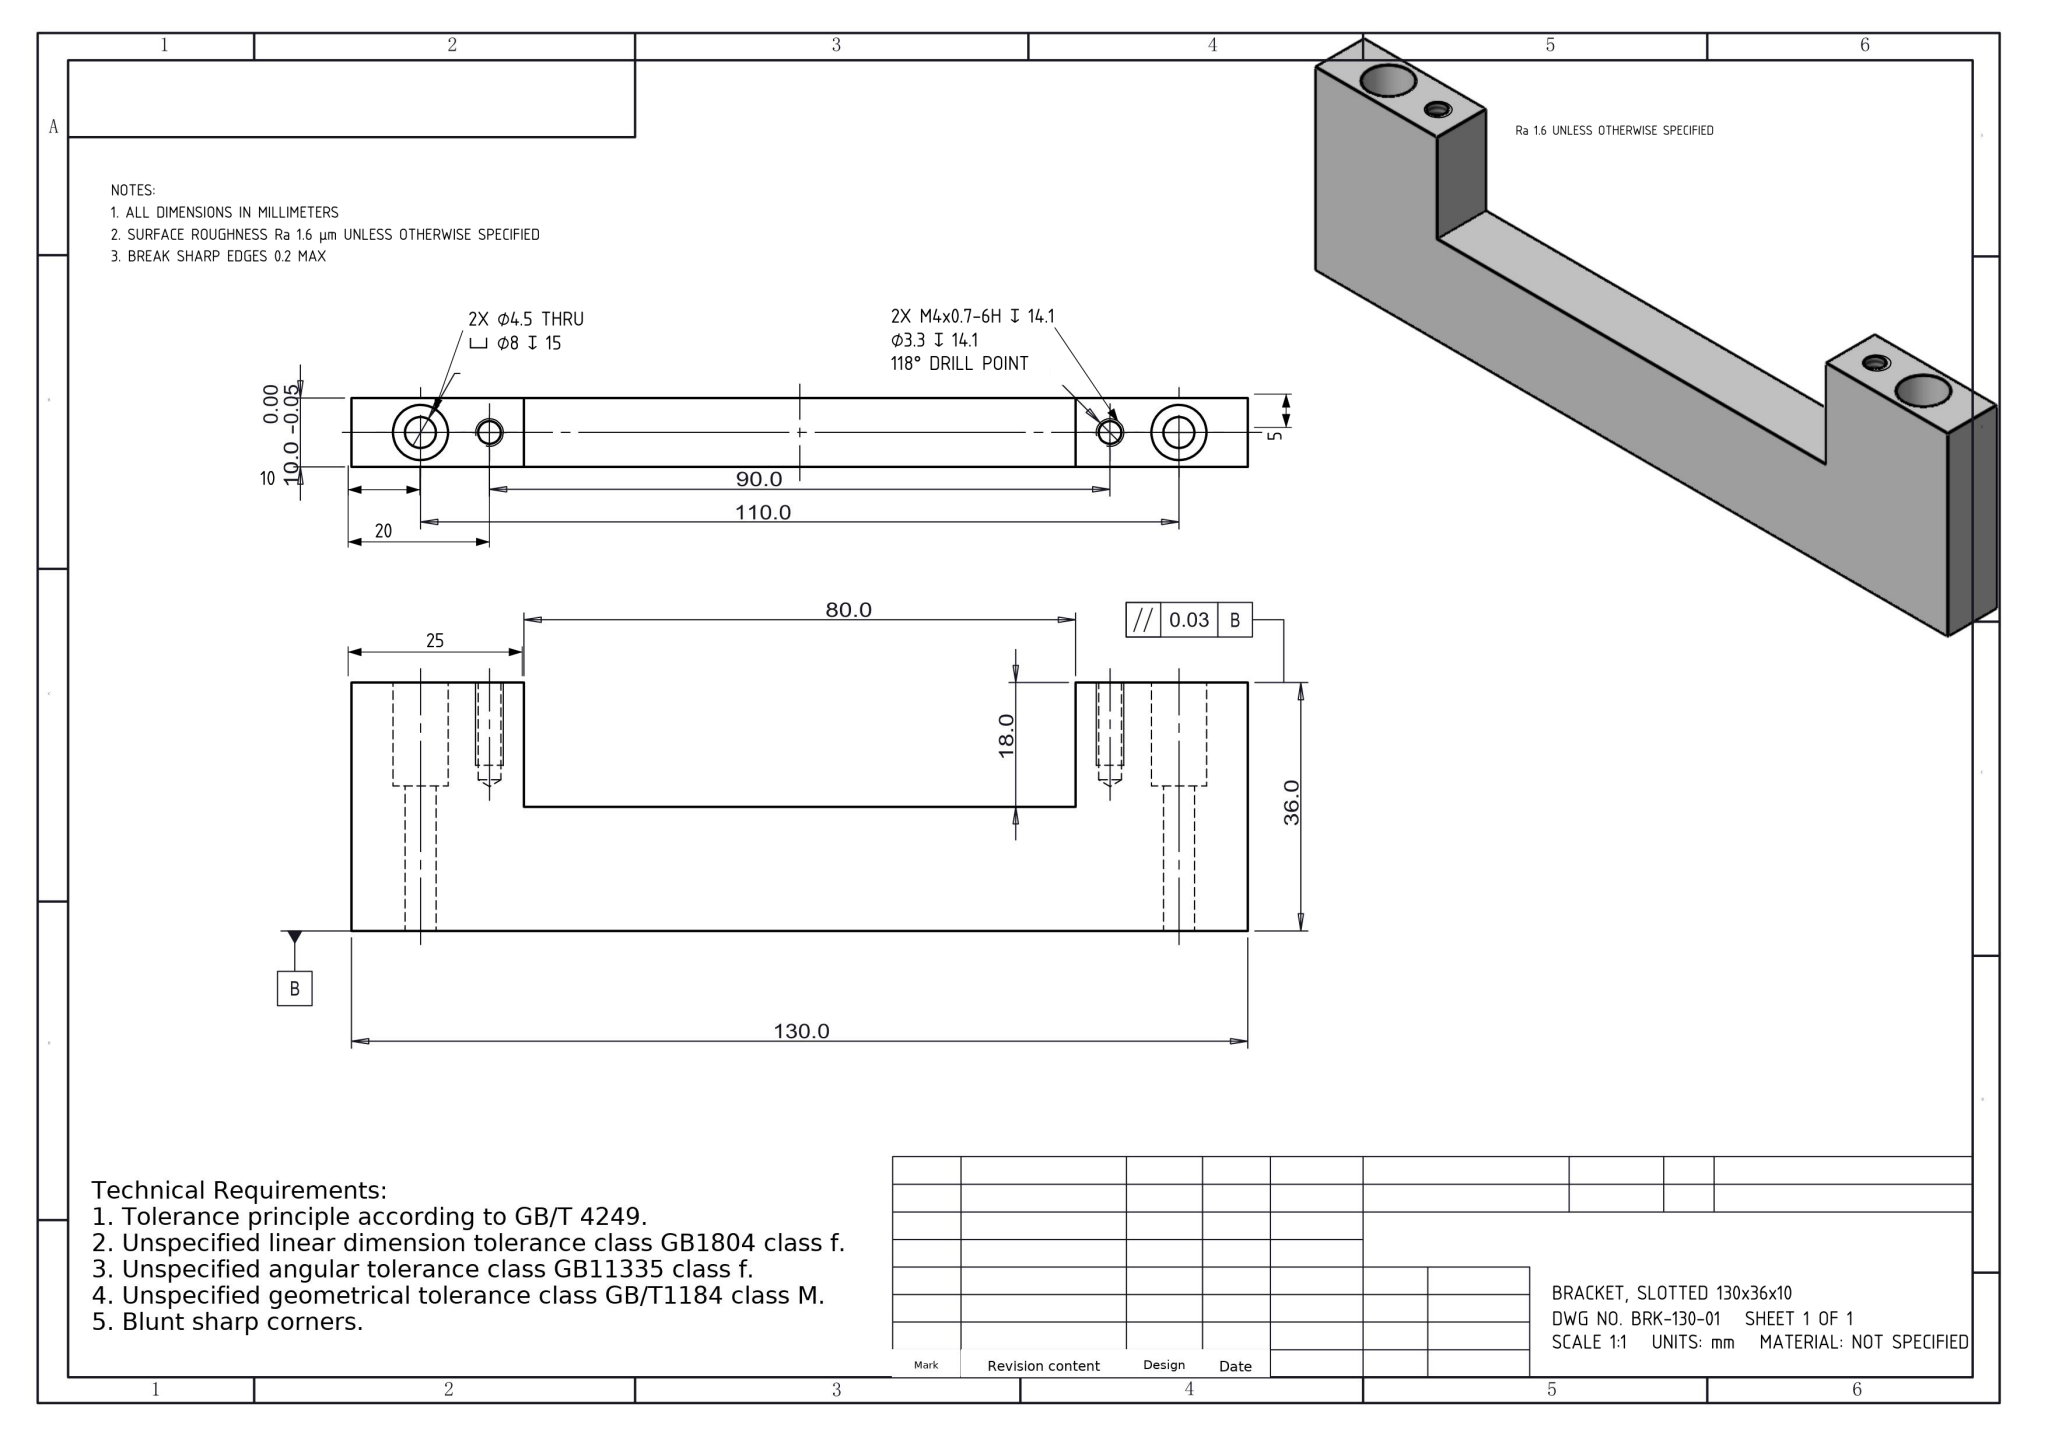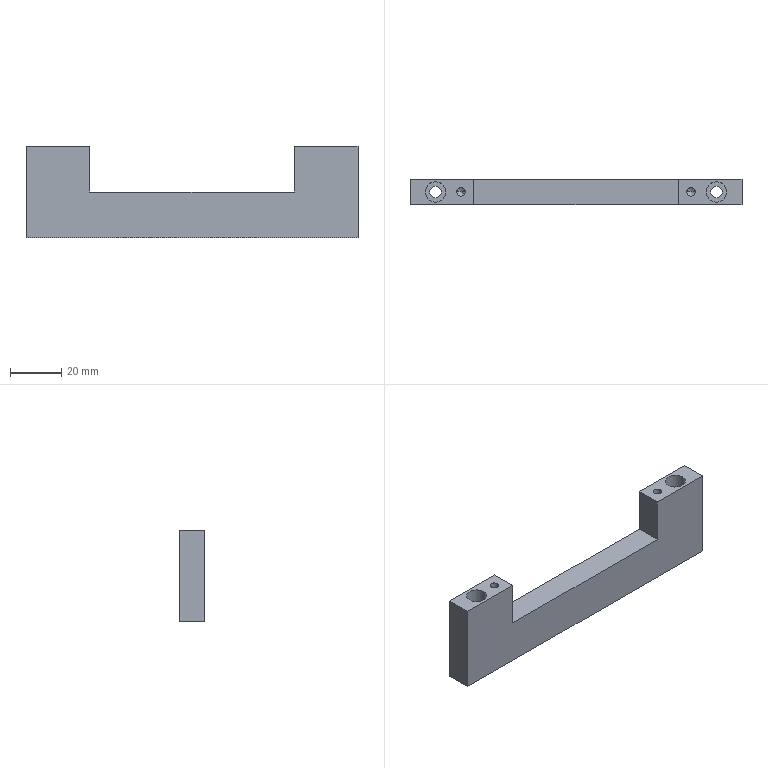Part | NX | mm | 1 solid | 28 faces | box 130 x 10 x 36 mm | volume 29977 mm3 | cylinder 12 | plane 12 | cone 4 | commonest cylinder face diameters 8 x4 4.5 x4 3.3 x4
STEP:
#1=COLOUR_RGB('',0.7529,0.7529,0.7529);
#2=FILL_AREA_STYLE_COLOUR('',#1);
#3=FILL_AREA_STYLE('',(#2));
#4=SURFACE_STYLE_FILL_AREA(#3);
#5=SURFACE_SIDE_STYLE('',(#4));
#6=SURFACE_STYLE_USAGE(.BOTH.,#5);
#7=PRESENTATION_STYLE_ASSIGNMENT((#6));
#8=CARTESIAN_POINT('',(51.,0.,21.));
#9=VERTEX_POINT('',#8);
#10=CARTESIAN_POINT('',(59.,0.,21.));
#11=VERTEX_POINT('',#10);
#12=CARTESIAN_POINT('',(55.,0.,21.));
#13=DIRECTION('',(0.,0.,1.));
#14=DIRECTION('',(1.,0.,0.));
#15=AXIS2_PLACEMENT_3D('',#12,#13,#14);
#16=CIRCLE('',#15,4.);
#17=EDGE_CURVE('',#9,#11,#16,.T.);
#18=ORIENTED_EDGE('',*,*,#17,.F.);
#19=CARTESIAN_POINT('',(51.,0.,36.));
#20=VERTEX_POINT('',#19);
#21=CARTESIAN_POINT('',(51.,0.,36.));
#22=DIRECTION('',(0.,0.,1.));
#23=VECTOR('',#22,1000.);
#24=LINE('',#21,#23);
#25=EDGE_CURVE('',#9,#20,#24,.T.);
#26=ORIENTED_EDGE('',*,*,#25,.T.);
#27=CARTESIAN_POINT('',(59.,0.,36.));
#28=VERTEX_POINT('',#27);
#29=CARTESIAN_POINT('',(55.,0.,36.));
#30=DIRECTION('',(0.,0.,1.));
#31=DIRECTION('',(1.,0.,0.));
#32=AXIS2_PLACEMENT_3D('',#29,#30,#31);
#33=CIRCLE('',#32,4.);
#34=EDGE_CURVE('',#20,#28,#33,.T.);
#35=ORIENTED_EDGE('',*,*,#34,.T.);
#36=CARTESIAN_POINT('',(59.,0.,36.));
#37=DIRECTION('',(0.,0.,1.));
#38=VECTOR('',#37,1000.);
#39=LINE('',#36,#38);
#40=EDGE_CURVE('',#11,#28,#39,.T.);
#41=ORIENTED_EDGE('',*,*,#40,.F.);
#42=EDGE_LOOP('',(#18,#26,#35,#41));
#43=FACE_OUTER_BOUND('',#42,.T.);
#44=CARTESIAN_POINT('',(55.,0.,36.));
#45=DIRECTION('',(0.,0.,1.));
#46=DIRECTION('',(1.,0.,0.));
#47=AXIS2_PLACEMENT_3D('',#44,#45,#46);
#48=CYLINDRICAL_SURFACE('',#47,4.);
#49=ADVANCED_FACE('',(#43),#48,.F.);
#50=CARTESIAN_POINT('',(52.75,0.,0.));
#51=VERTEX_POINT('',#50);
#52=CARTESIAN_POINT('',(57.25,0.,0.));
#53=VERTEX_POINT('',#52);
#54=CARTESIAN_POINT('',(55.,0.,0.));
#55=DIRECTION('',(0.,0.,1.));
#56=DIRECTION('',(1.,0.,0.));
#57=AXIS2_PLACEMENT_3D('',#54,#55,#56);
#58=CIRCLE('',#57,2.25);
#59=EDGE_CURVE('',#51,#53,#58,.T.);
#60=ORIENTED_EDGE('',*,*,#59,.F.);
#61=CARTESIAN_POINT('',(52.75,0.,21.));
#62=VERTEX_POINT('',#61);
#63=CARTESIAN_POINT('',(52.75,0.,36.));
#64=DIRECTION('',(0.,0.,1.));
#65=VECTOR('',#64,1000.);
#66=LINE('',#63,#65);
#67=EDGE_CURVE('',#51,#62,#66,.T.);
#68=ORIENTED_EDGE('',*,*,#67,.T.);
#69=CARTESIAN_POINT('',(57.25,0.,21.));
#70=VERTEX_POINT('',#69);
#71=CARTESIAN_POINT('',(55.,0.,21.));
#72=DIRECTION('',(0.,0.,1.));
#73=DIRECTION('',(1.,0.,0.));
#74=AXIS2_PLACEMENT_3D('',#71,#72,#73);
#75=CIRCLE('',#74,2.25);
#76=EDGE_CURVE('',#62,#70,#75,.T.);
#77=ORIENTED_EDGE('',*,*,#76,.T.);
#78=CARTESIAN_POINT('',(57.25,0.,36.));
#79=DIRECTION('',(0.,0.,1.));
#80=VECTOR('',#79,1000.);
#81=LINE('',#78,#80);
#82=EDGE_CURVE('',#53,#70,#81,.T.);
#83=ORIENTED_EDGE('',*,*,#82,.F.);
#84=EDGE_LOOP('',(#60,#68,#77,#83));
#85=FACE_OUTER_BOUND('',#84,.T.);
#86=CARTESIAN_POINT('',(55.,0.,36.));
#87=DIRECTION('',(0.,0.,1.));
#88=DIRECTION('',(1.,0.,0.));
#89=AXIS2_PLACEMENT_3D('',#86,#87,#88);
#90=CYLINDRICAL_SURFACE('',#89,2.25);
#91=ADVANCED_FACE('',(#85),#90,.F.);
#92=CARTESIAN_POINT('',(-59.,0.,21.));
#93=VERTEX_POINT('',#92);
#94=CARTESIAN_POINT('',(-51.,0.,21.));
#95=VERTEX_POINT('',#94);
#96=CARTESIAN_POINT('',(-55.,0.,21.));
#97=DIRECTION('',(0.,0.,1.));
#98=DIRECTION('',(1.,0.,0.));
#99=AXIS2_PLACEMENT_3D('',#96,#97,#98);
#100=CIRCLE('',#99,4.);
#101=EDGE_CURVE('',#93,#95,#100,.T.);
#102=ORIENTED_EDGE('',*,*,#101,.F.);
#103=CARTESIAN_POINT('',(-59.,0.,36.));
#104=VERTEX_POINT('',#103);
#105=CARTESIAN_POINT('',(-59.,0.,36.));
#106=DIRECTION('',(0.,0.,1.));
#107=VECTOR('',#106,1000.);
#108=LINE('',#105,#107);
#109=EDGE_CURVE('',#93,#104,#108,.T.);
#110=ORIENTED_EDGE('',*,*,#109,.T.);
#111=CARTESIAN_POINT('',(-51.,0.,36.));
#112=VERTEX_POINT('',#111);
#113=CARTESIAN_POINT('',(-55.,0.,36.));
#114=DIRECTION('',(0.,0.,1.));
#115=DIRECTION('',(1.,0.,0.));
#116=AXIS2_PLACEMENT_3D('',#113,#114,#115);
#117=CIRCLE('',#116,4.);
#118=EDGE_CURVE('',#104,#112,#117,.T.);
#119=ORIENTED_EDGE('',*,*,#118,.T.);
#120=CARTESIAN_POINT('',(-51.,0.,36.));
#121=DIRECTION('',(0.,0.,1.));
#122=VECTOR('',#121,1000.);
#123=LINE('',#120,#122);
#124=EDGE_CURVE('',#95,#112,#123,.T.);
#125=ORIENTED_EDGE('',*,*,#124,.F.);
#126=EDGE_LOOP('',(#102,#110,#119,#125));
#127=FACE_OUTER_BOUND('',#126,.T.);
#128=CARTESIAN_POINT('',(-55.,0.,36.));
#129=DIRECTION('',(0.,0.,1.));
#130=DIRECTION('',(1.,0.,0.));
#131=AXIS2_PLACEMENT_3D('',#128,#129,#130);
#132=CYLINDRICAL_SURFACE('',#131,4.);
#133=ADVANCED_FACE('',(#127),#132,.F.);
#134=CARTESIAN_POINT('',(-57.25,0.,0.));
#135=VERTEX_POINT('',#134);
#136=CARTESIAN_POINT('',(-52.75,0.,0.));
#137=VERTEX_POINT('',#136);
#138=CARTESIAN_POINT('',(-55.,0.,0.));
#139=DIRECTION('',(0.,0.,1.));
#140=DIRECTION('',(1.,0.,0.));
#141=AXIS2_PLACEMENT_3D('',#138,#139,#140);
#142=CIRCLE('',#141,2.25);
#143=EDGE_CURVE('',#135,#137,#142,.T.);
#144=ORIENTED_EDGE('',*,*,#143,.F.);
#145=CARTESIAN_POINT('',(-57.25,0.,21.));
#146=VERTEX_POINT('',#145);
#147=CARTESIAN_POINT('',(-57.25,0.,36.));
#148=DIRECTION('',(0.,0.,1.));
#149=VECTOR('',#148,1000.);
#150=LINE('',#147,#149);
#151=EDGE_CURVE('',#135,#146,#150,.T.);
#152=ORIENTED_EDGE('',*,*,#151,.T.);
#153=CARTESIAN_POINT('',(-52.75,0.,21.));
#154=VERTEX_POINT('',#153);
#155=CARTESIAN_POINT('',(-55.,0.,21.));
#156=DIRECTION('',(0.,0.,1.));
#157=DIRECTION('',(1.,0.,0.));
#158=AXIS2_PLACEMENT_3D('',#155,#156,#157);
#159=CIRCLE('',#158,2.25);
#160=EDGE_CURVE('',#146,#154,#159,.T.);
#161=ORIENTED_EDGE('',*,*,#160,.T.);
#162=CARTESIAN_POINT('',(-52.75,0.,36.));
#163=DIRECTION('',(0.,0.,1.));
#164=VECTOR('',#163,1000.);
#165=LINE('',#162,#164);
#166=EDGE_CURVE('',#137,#154,#165,.T.);
#167=ORIENTED_EDGE('',*,*,#166,.F.);
#168=EDGE_LOOP('',(#144,#152,#161,#167));
#169=FACE_OUTER_BOUND('',#168,.T.);
#170=CARTESIAN_POINT('',(-55.,0.,36.));
#171=DIRECTION('',(0.,0.,1.));
#172=DIRECTION('',(1.,0.,0.));
#173=AXIS2_PLACEMENT_3D('',#170,#171,#172);
#174=CYLINDRICAL_SURFACE('',#173,2.25);
#175=ADVANCED_FACE('',(#169),#174,.F.);
#176=CARTESIAN_POINT('',(43.35,0.,21.9));
#177=VERTEX_POINT('',#176);
#178=CARTESIAN_POINT('',(46.65,0.,21.9));
#179=VERTEX_POINT('',#178);
#180=CARTESIAN_POINT('',(45.,0.,21.9));
#181=DIRECTION('',(0.,0.,1.));
#182=DIRECTION('',(1.,0.,0.));
#183=AXIS2_PLACEMENT_3D('',#180,#181,#182);
#184=CIRCLE('',#183,1.65);
#185=EDGE_CURVE('',#177,#179,#184,.T.);
#186=ORIENTED_EDGE('',*,*,#185,.F.);
#187=CARTESIAN_POINT('',(43.35,0.,36.));
#188=VERTEX_POINT('',#187);
#189=CARTESIAN_POINT('',(43.35,0.,36.));
#190=DIRECTION('',(0.,0.,1.));
#191=VECTOR('',#190,1000.);
#192=LINE('',#189,#191);
#193=EDGE_CURVE('',#177,#188,#192,.T.);
#194=ORIENTED_EDGE('',*,*,#193,.T.);
#195=CARTESIAN_POINT('',(46.65,0.,36.));
#196=VERTEX_POINT('',#195);
#197=CARTESIAN_POINT('',(45.,0.,36.));
#198=DIRECTION('',(0.,0.,1.));
#199=DIRECTION('',(1.,0.,0.));
#200=AXIS2_PLACEMENT_3D('',#197,#198,#199);
#201=CIRCLE('',#200,1.65);
#202=EDGE_CURVE('',#188,#196,#201,.T.);
#203=ORIENTED_EDGE('',*,*,#202,.T.);
#204=CARTESIAN_POINT('',(46.65,0.,36.));
#205=DIRECTION('',(0.,0.,1.));
#206=VECTOR('',#205,1000.);
#207=LINE('',#204,#206);
#208=EDGE_CURVE('',#179,#196,#207,.T.);
#209=ORIENTED_EDGE('',*,*,#208,.F.);
#210=EDGE_LOOP('',(#186,#194,#203,#209));
#211=FACE_OUTER_BOUND('',#210,.T.);
#212=CARTESIAN_POINT('',(45.,0.,36.));
#213=DIRECTION('',(0.,0.,1.));
#214=DIRECTION('',(1.,0.,0.));
#215=AXIS2_PLACEMENT_3D('',#212,#213,#214);
#216=CYLINDRICAL_SURFACE('',#215,1.65);
#217=ADVANCED_FACE('',(#211),#216,.F.);
#218=CARTESIAN_POINT('',(45.,0.,20.909));
#219=VERTEX_POINT('',#218);
#220=CARTESIAN_POINT('',(46.65,0.,21.9));
#221=DIRECTION('',(0.8572,0.,0.515));
#222=VECTOR('',#221,1000.);
#223=LINE('',#220,#222);
#224=EDGE_CURVE('',#219,#179,#223,.T.);
#225=ORIENTED_EDGE('',*,*,#224,.F.);
#226=CARTESIAN_POINT('',(43.35,0.,21.9));
#227=DIRECTION('',(-0.8572,0.,0.515));
#228=VECTOR('',#227,1000.);
#229=LINE('',#226,#228);
#230=EDGE_CURVE('',#219,#177,#229,.T.);
#231=ORIENTED_EDGE('',*,*,#230,.T.);
#232=ORIENTED_EDGE('',*,*,#185,.T.);
#233=EDGE_LOOP('',(#225,#231,#232));
#234=FACE_OUTER_BOUND('',#233,.T.);
#235=CARTESIAN_POINT('',(45.,0.,21.9));
#236=DIRECTION('',(0.,0.,1.));
#237=DIRECTION('',(1.,0.,0.));
#238=AXIS2_PLACEMENT_3D('',#235,#236,#237);
#239=CONICAL_SURFACE('',#238,1.65,1.03);
#240=ADVANCED_FACE('',(#234),#239,.F.);
#241=CARTESIAN_POINT('',(-46.65,0.,21.9));
#242=VERTEX_POINT('',#241);
#243=CARTESIAN_POINT('',(-43.35,0.,21.9));
#244=VERTEX_POINT('',#243);
#245=CARTESIAN_POINT('',(-45.,0.,21.9));
#246=DIRECTION('',(0.,0.,1.));
#247=DIRECTION('',(1.,0.,0.));
#248=AXIS2_PLACEMENT_3D('',#245,#246,#247);
#249=CIRCLE('',#248,1.65);
#250=EDGE_CURVE('',#242,#244,#249,.T.);
#251=ORIENTED_EDGE('',*,*,#250,.F.);
#252=CARTESIAN_POINT('',(-46.65,0.,36.));
#253=VERTEX_POINT('',#252);
#254=CARTESIAN_POINT('',(-46.65,0.,36.));
#255=DIRECTION('',(0.,0.,1.));
#256=VECTOR('',#255,1000.);
#257=LINE('',#254,#256);
#258=EDGE_CURVE('',#242,#253,#257,.T.);
#259=ORIENTED_EDGE('',*,*,#258,.T.);
#260=CARTESIAN_POINT('',(-43.35,0.,36.));
#261=VERTEX_POINT('',#260);
#262=CARTESIAN_POINT('',(-45.,0.,36.));
#263=DIRECTION('',(0.,0.,1.));
#264=DIRECTION('',(1.,0.,0.));
#265=AXIS2_PLACEMENT_3D('',#262,#263,#264);
#266=CIRCLE('',#265,1.65);
#267=EDGE_CURVE('',#253,#261,#266,.T.);
#268=ORIENTED_EDGE('',*,*,#267,.T.);
#269=CARTESIAN_POINT('',(-43.35,0.,36.));
#270=DIRECTION('',(0.,0.,1.));
#271=VECTOR('',#270,1000.);
#272=LINE('',#269,#271);
#273=EDGE_CURVE('',#244,#261,#272,.T.);
#274=ORIENTED_EDGE('',*,*,#273,.F.);
#275=EDGE_LOOP('',(#251,#259,#268,#274));
#276=FACE_OUTER_BOUND('',#275,.T.);
#277=CARTESIAN_POINT('',(-45.,0.,36.));
#278=DIRECTION('',(0.,0.,1.));
#279=DIRECTION('',(1.,0.,0.));
#280=AXIS2_PLACEMENT_3D('',#277,#278,#279);
#281=CYLINDRICAL_SURFACE('',#280,1.65);
#282=ADVANCED_FACE('',(#276),#281,.F.);
#283=CARTESIAN_POINT('',(-45.,0.,20.909));
#284=VERTEX_POINT('',#283);
#285=CARTESIAN_POINT('',(-43.35,0.,21.9));
#286=DIRECTION('',(0.8572,0.,0.515));
#287=VECTOR('',#286,1000.);
#288=LINE('',#285,#287);
#289=EDGE_CURVE('',#284,#244,#288,.T.);
#290=ORIENTED_EDGE('',*,*,#289,.F.);
#291=CARTESIAN_POINT('',(-46.65,0.,21.9));
#292=DIRECTION('',(-0.8572,0.,0.515));
#293=VECTOR('',#292,1000.);
#294=LINE('',#291,#293);
#295=EDGE_CURVE('',#284,#242,#294,.T.);
#296=ORIENTED_EDGE('',*,*,#295,.T.);
#297=ORIENTED_EDGE('',*,*,#250,.T.);
#298=EDGE_LOOP('',(#290,#296,#297));
#299=FACE_OUTER_BOUND('',#298,.T.);
#300=CARTESIAN_POINT('',(-45.,0.,21.9));
#301=DIRECTION('',(0.,0.,1.));
#302=DIRECTION('',(1.,0.,0.));
#303=AXIS2_PLACEMENT_3D('',#300,#301,#302);
#304=CONICAL_SURFACE('',#303,1.65,1.03);
#305=ADVANCED_FACE('',(#299),#304,.F.);
#306=CARTESIAN_POINT('',(-40.,5.,36.));
#307=VERTEX_POINT('',#306);
#308=CARTESIAN_POINT('',(-40.,-5.,36.));
#309=VERTEX_POINT('',#308);
#310=CARTESIAN_POINT('',(-40.,5.,36.));
#311=DIRECTION('',(0.,-1.,0.));
#312=VECTOR('',#311,1000.);
#313=LINE('',#310,#312);
#314=EDGE_CURVE('',#307,#309,#313,.T.);
#315=ORIENTED_EDGE('',*,*,#314,.F.);
#316=CARTESIAN_POINT('',(-65.,5.,36.));
#317=VERTEX_POINT('',#316);
#318=CARTESIAN_POINT('',(-65.,5.,36.));
#319=DIRECTION('',(-1.,0.,0.));
#320=VECTOR('',#319,1000.);
#321=LINE('',#318,#320);
#322=EDGE_CURVE('',#307,#317,#321,.T.);
#323=ORIENTED_EDGE('',*,*,#322,.T.);
#324=CARTESIAN_POINT('',(-65.,-5.,36.));
#325=VERTEX_POINT('',#324);
#326=CARTESIAN_POINT('',(-65.,5.,36.));
#327=DIRECTION('',(0.,-1.,0.));
#328=VECTOR('',#327,1000.);
#329=LINE('',#326,#328);
#330=EDGE_CURVE('',#317,#325,#329,.T.);
#331=ORIENTED_EDGE('',*,*,#330,.T.);
#332=CARTESIAN_POINT('',(-65.,-5.,36.));
#333=DIRECTION('',(1.,0.,0.));
#334=VECTOR('',#333,1000.);
#335=LINE('',#332,#334);
#336=EDGE_CURVE('',#325,#309,#335,.T.);
#337=ORIENTED_EDGE('',*,*,#336,.T.);
#338=EDGE_LOOP('',(#315,#323,#331,#337));
#339=FACE_OUTER_BOUND('',#338,.T.);
#340=CARTESIAN_POINT('',(-45.,0.,36.));
#341=DIRECTION('',(0.,0.,1.));
#342=DIRECTION('',(1.,0.,0.));
#343=AXIS2_PLACEMENT_3D('',#340,#341,#342);
#344=CIRCLE('',#343,1.65);
#345=EDGE_CURVE('',#261,#253,#344,.T.);
#346=ORIENTED_EDGE('',*,*,#345,.F.);
#347=ORIENTED_EDGE('',*,*,#267,.F.);
#348=EDGE_LOOP('',(#346,#347));
#349=FACE_BOUND('',#348,.T.);
#350=CARTESIAN_POINT('',(-55.,0.,36.));
#351=DIRECTION('',(0.,0.,1.));
#352=DIRECTION('',(1.,0.,0.));
#353=AXIS2_PLACEMENT_3D('',#350,#351,#352);
#354=CIRCLE('',#353,4.);
#355=EDGE_CURVE('',#112,#104,#354,.T.);
#356=ORIENTED_EDGE('',*,*,#355,.F.);
#357=ORIENTED_EDGE('',*,*,#118,.F.);
#358=EDGE_LOOP('',(#356,#357));
#359=FACE_BOUND('',#358,.T.);
#360=CARTESIAN_POINT('',(65.,-5.,36.));
#361=DIRECTION('',(0.,0.,1.));
#362=DIRECTION('',(1.,0.,0.));
#363=AXIS2_PLACEMENT_3D('',#360,#361,#362);
#364=PLANE('',#363);
#365=ADVANCED_FACE('',(#339,#349,#359),#364,.T.);
#366=CARTESIAN_POINT('',(65.,-5.,0.));
#367=VERTEX_POINT('',#366);
#368=CARTESIAN_POINT('',(65.,5.,0.));
#369=VERTEX_POINT('',#368);
#370=CARTESIAN_POINT('',(65.,5.,0.));
#371=DIRECTION('',(0.,1.,0.));
#372=VECTOR('',#371,1000.);
#373=LINE('',#370,#372);
#374=EDGE_CURVE('',#367,#369,#373,.T.);
#375=ORIENTED_EDGE('',*,*,#374,.T.);
#376=CARTESIAN_POINT('',(65.,5.,36.));
#377=VERTEX_POINT('',#376);
#378=CARTESIAN_POINT('',(65.,5.,36.));
#379=DIRECTION('',(0.,0.,-1.));
#380=VECTOR('',#379,1000.);
#381=LINE('',#378,#380);
#382=EDGE_CURVE('',#377,#369,#381,.T.);
#383=ORIENTED_EDGE('',*,*,#382,.F.);
#384=CARTESIAN_POINT('',(65.,-5.,36.));
#385=VERTEX_POINT('',#384);
#386=CARTESIAN_POINT('',(65.,5.,36.));
#387=DIRECTION('',(0.,1.,0.));
#388=VECTOR('',#387,1000.);
#389=LINE('',#386,#388);
#390=EDGE_CURVE('',#385,#377,#389,.T.);
#391=ORIENTED_EDGE('',*,*,#390,.F.);
#392=CARTESIAN_POINT('',(65.,-5.,36.));
#393=DIRECTION('',(0.,0.,-1.));
#394=VECTOR('',#393,1000.);
#395=LINE('',#392,#394);
#396=EDGE_CURVE('',#385,#367,#395,.T.);
#397=ORIENTED_EDGE('',*,*,#396,.T.);
#398=EDGE_LOOP('',(#375,#383,#391,#397));
#399=FACE_OUTER_BOUND('',#398,.T.);
#400=CARTESIAN_POINT('',(65.,5.,36.));
#401=DIRECTION('',(-1.,0.,0.));
#402=DIRECTION('',(0.,0.,1.));
#403=AXIS2_PLACEMENT_3D('',#400,#401,#402);
#404=PLANE('',#403);
#405=ADVANCED_FACE('',(#399),#404,.F.);
#406=ORIENTED_EDGE('',*,*,#322,.F.);
#407=CARTESIAN_POINT('',(-40.,5.,18.));
#408=VERTEX_POINT('',#407);
#409=CARTESIAN_POINT('',(-40.,5.,18.));
#410=DIRECTION('',(0.,0.,1.));
#411=VECTOR('',#410,1000.);
#412=LINE('',#409,#411);
#413=EDGE_CURVE('',#408,#307,#412,.T.);
#414=ORIENTED_EDGE('',*,*,#413,.F.);
#415=CARTESIAN_POINT('',(40.,5.,18.));
#416=VERTEX_POINT('',#415);
#417=CARTESIAN_POINT('',(-40.,5.,18.));
#418=DIRECTION('',(-1.,0.,0.));
#419=VECTOR('',#418,1000.);
#420=LINE('',#417,#419);
#421=EDGE_CURVE('',#416,#408,#420,.T.);
#422=ORIENTED_EDGE('',*,*,#421,.F.);
#423=CARTESIAN_POINT('',(40.,5.,36.));
#424=VERTEX_POINT('',#423);
#425=CARTESIAN_POINT('',(40.,5.,18.));
#426=DIRECTION('',(0.,0.,1.));
#427=VECTOR('',#426,1000.);
#428=LINE('',#425,#427);
#429=EDGE_CURVE('',#416,#424,#428,.T.);
#430=ORIENTED_EDGE('',*,*,#429,.T.);
#431=CARTESIAN_POINT('',(-65.,5.,36.));
#432=DIRECTION('',(-1.,0.,0.));
#433=VECTOR('',#432,1000.);
#434=LINE('',#431,#433);
#435=EDGE_CURVE('',#377,#424,#434,.T.);
#436=ORIENTED_EDGE('',*,*,#435,.F.);
#437=ORIENTED_EDGE('',*,*,#382,.T.);
#438=CARTESIAN_POINT('',(-65.,5.,0.));
#439=VERTEX_POINT('',#438);
#440=CARTESIAN_POINT('',(-65.,5.,0.));
#441=DIRECTION('',(-1.,0.,0.));
#442=VECTOR('',#441,1000.);
#443=LINE('',#440,#442);
#444=EDGE_CURVE('',#369,#439,#443,.T.);
#445=ORIENTED_EDGE('',*,*,#444,.T.);
#446=CARTESIAN_POINT('',(-65.,5.,36.));
#447=DIRECTION('',(0.,0.,-1.));
#448=VECTOR('',#447,1000.);
#449=LINE('',#446,#448);
#450=EDGE_CURVE('',#317,#439,#449,.T.);
#451=ORIENTED_EDGE('',*,*,#450,.F.);
#452=EDGE_LOOP('',(#406,#414,#422,#430,#436,#437,#445,#451));
#453=FACE_OUTER_BOUND('',#452,.T.);
#454=CARTESIAN_POINT('',(-65.,5.,36.));
#455=DIRECTION('',(-0.,-1.,0.));
#456=DIRECTION('',(1.,-0.,0.));
#457=AXIS2_PLACEMENT_3D('',#454,#455,#456);
#458=PLANE('',#457);
#459=ADVANCED_FACE('',(#453),#458,.F.);
#460=CARTESIAN_POINT('',(-65.,-5.,0.));
#461=VERTEX_POINT('',#460);
#462=CARTESIAN_POINT('',(-65.,5.,0.));
#463=DIRECTION('',(0.,-1.,0.));
#464=VECTOR('',#463,1000.);
#465=LINE('',#462,#464);
#466=EDGE_CURVE('',#439,#461,#465,.T.);
#467=ORIENTED_EDGE('',*,*,#466,.T.);
#468=CARTESIAN_POINT('',(-65.,-5.,36.));
#469=DIRECTION('',(0.,0.,-1.));
#470=VECTOR('',#469,1000.);
#471=LINE('',#468,#470);
#472=EDGE_CURVE('',#325,#461,#471,.T.);
#473=ORIENTED_EDGE('',*,*,#472,.F.);
#474=ORIENTED_EDGE('',*,*,#330,.F.);
#475=ORIENTED_EDGE('',*,*,#450,.T.);
#476=EDGE_LOOP('',(#467,#473,#474,#475));
#477=FACE_OUTER_BOUND('',#476,.T.);
#478=CARTESIAN_POINT('',(-65.,5.,36.));
#479=DIRECTION('',(1.,0.,0.));
#480=DIRECTION('',(0.,0.,-1.));
#481=AXIS2_PLACEMENT_3D('',#478,#479,#480);
#482=PLANE('',#481);
#483=ADVANCED_FACE('',(#477),#482,.F.);
#484=CARTESIAN_POINT('',(-40.,-5.,18.));
#485=VERTEX_POINT('',#484);
#486=CARTESIAN_POINT('',(40.,-5.,18.));
#487=VERTEX_POINT('',#486);
#488=CARTESIAN_POINT('',(-40.,-5.,18.));
#489=DIRECTION('',(1.,0.,0.));
#490=VECTOR('',#489,1000.);
#491=LINE('',#488,#490);
#492=EDGE_CURVE('',#485,#487,#491,.T.);
#493=ORIENTED_EDGE('',*,*,#492,.F.);
#494=CARTESIAN_POINT('',(-40.,-5.,18.));
#495=DIRECTION('',(0.,0.,1.));
#496=VECTOR('',#495,1000.);
#497=LINE('',#494,#496);
#498=EDGE_CURVE('',#485,#309,#497,.T.);
#499=ORIENTED_EDGE('',*,*,#498,.T.);
#500=ORIENTED_EDGE('',*,*,#336,.F.);
#501=ORIENTED_EDGE('',*,*,#472,.T.);
#502=CARTESIAN_POINT('',(-65.,-5.,0.));
#503=DIRECTION('',(1.,0.,0.));
#504=VECTOR('',#503,1000.);
#505=LINE('',#502,#504);
#506=EDGE_CURVE('',#461,#367,#505,.T.);
#507=ORIENTED_EDGE('',*,*,#506,.T.);
#508=ORIENTED_EDGE('',*,*,#396,.F.);
#509=CARTESIAN_POINT('',(40.,-5.,36.));
#510=VERTEX_POINT('',#509);
#511=CARTESIAN_POINT('',(-65.,-5.,36.));
#512=DIRECTION('',(1.,0.,0.));
#513=VECTOR('',#512,1000.);
#514=LINE('',#511,#513);
#515=EDGE_CURVE('',#510,#385,#514,.T.);
#516=ORIENTED_EDGE('',*,*,#515,.F.);
#517=CARTESIAN_POINT('',(40.,-5.,18.));
#518=DIRECTION('',(0.,0.,1.));
#519=VECTOR('',#518,1000.);
#520=LINE('',#517,#519);
#521=EDGE_CURVE('',#487,#510,#520,.T.);
#522=ORIENTED_EDGE('',*,*,#521,.F.);
#523=EDGE_LOOP('',(#493,#499,#500,#501,#507,#508,#516,#522));
#524=FACE_OUTER_BOUND('',#523,.T.);
#525=CARTESIAN_POINT('',(-65.,-5.,36.));
#526=DIRECTION('',(0.,1.,0.));
#527=DIRECTION('',(0.,0.,1.));
#528=AXIS2_PLACEMENT_3D('',#525,#526,#527);
#529=PLANE('',#528);
#530=ADVANCED_FACE('',(#524),#529,.F.);
#531=CARTESIAN_POINT('',(40.,5.,36.));
#532=DIRECTION('',(0.,1.,0.));
#533=VECTOR('',#532,1000.);
#534=LINE('',#531,#533);
#535=EDGE_CURVE('',#510,#424,#534,.T.);
#536=ORIENTED_EDGE('',*,*,#535,.F.);
#537=ORIENTED_EDGE('',*,*,#515,.T.);
#538=ORIENTED_EDGE('',*,*,#390,.T.);
#539=ORIENTED_EDGE('',*,*,#435,.T.);
#540=EDGE_LOOP('',(#536,#537,#538,#539));
#541=FACE_OUTER_BOUND('',#540,.T.);
#542=CARTESIAN_POINT('',(55.,0.,36.));
#543=DIRECTION('',(0.,0.,1.));
#544=DIRECTION('',(1.,0.,0.));
#545=AXIS2_PLACEMENT_3D('',#542,#543,#544);
#546=CIRCLE('',#545,4.);
#547=EDGE_CURVE('',#28,#20,#546,.T.);
#548=ORIENTED_EDGE('',*,*,#547,.F.);
#549=ORIENTED_EDGE('',*,*,#34,.F.);
#550=EDGE_LOOP('',(#548,#549));
#551=FACE_BOUND('',#550,.T.);
#552=CARTESIAN_POINT('',(45.,0.,36.));
#553=DIRECTION('',(0.,0.,1.));
#554=DIRECTION('',(1.,0.,0.));
#555=AXIS2_PLACEMENT_3D('',#552,#553,#554);
#556=CIRCLE('',#555,1.65);
#557=EDGE_CURVE('',#196,#188,#556,.T.);
#558=ORIENTED_EDGE('',*,*,#557,.F.);
#559=ORIENTED_EDGE('',*,*,#202,.F.);
#560=EDGE_LOOP('',(#558,#559));
#561=FACE_BOUND('',#560,.T.);
#562=CARTESIAN_POINT('',(65.,-5.,36.));
#563=DIRECTION('',(0.,0.,1.));
#564=DIRECTION('',(1.,0.,0.));
#565=AXIS2_PLACEMENT_3D('',#562,#563,#564);
#566=PLANE('',#565);
#567=ADVANCED_FACE('',(#541,#551,#561),#566,.T.);
#568=CARTESIAN_POINT('',(55.,0.,0.));
#569=DIRECTION('',(0.,0.,1.));
#570=DIRECTION('',(1.,0.,0.));
#571=AXIS2_PLACEMENT_3D('',#568,#569,#570);
#572=CIRCLE('',#571,2.25);
#573=EDGE_CURVE('',#53,#51,#572,.T.);
#574=ORIENTED_EDGE('',*,*,#573,.T.);
#575=ORIENTED_EDGE('',*,*,#59,.T.);
#576=EDGE_LOOP('',(#574,#575));
#577=FACE_BOUND('',#576,.T.);
#578=CARTESIAN_POINT('',(-55.,0.,0.));
#579=DIRECTION('',(0.,0.,1.));
#580=DIRECTION('',(1.,0.,0.));
#581=AXIS2_PLACEMENT_3D('',#578,#579,#580);
#582=CIRCLE('',#581,2.25);
#583=EDGE_CURVE('',#137,#135,#582,.T.);
#584=ORIENTED_EDGE('',*,*,#583,.T.);
#585=ORIENTED_EDGE('',*,*,#143,.T.);
#586=EDGE_LOOP('',(#584,#585));
#587=FACE_BOUND('',#586,.T.);
#588=ORIENTED_EDGE('',*,*,#374,.F.);
#589=ORIENTED_EDGE('',*,*,#506,.F.);
#590=ORIENTED_EDGE('',*,*,#466,.F.);
#591=ORIENTED_EDGE('',*,*,#444,.F.);
#592=EDGE_LOOP('',(#588,#589,#590,#591));
#593=FACE_OUTER_BOUND('',#592,.T.);
#594=CARTESIAN_POINT('',(65.,-5.,0.));
#595=DIRECTION('',(0.,0.,1.));
#596=DIRECTION('',(1.,0.,0.));
#597=AXIS2_PLACEMENT_3D('',#594,#595,#596);
#598=PLANE('',#597);
#599=ADVANCED_FACE('',(#577,#587,#593),#598,.F.);
#600=ORIENTED_EDGE('',*,*,#295,.F.);
#601=ORIENTED_EDGE('',*,*,#289,.T.);
#602=CARTESIAN_POINT('',(-45.,0.,21.9));
#603=DIRECTION('',(0.,0.,1.));
#604=DIRECTION('',(1.,0.,0.));
#605=AXIS2_PLACEMENT_3D('',#602,#603,#604);
#606=CIRCLE('',#605,1.65);
#607=EDGE_CURVE('',#244,#242,#606,.T.);
#608=ORIENTED_EDGE('',*,*,#607,.T.);
#609=EDGE_LOOP('',(#600,#601,#608));
#610=FACE_OUTER_BOUND('',#609,.T.);
#611=CARTESIAN_POINT('',(-45.,0.,21.9));
#612=DIRECTION('',(0.,0.,1.));
#613=DIRECTION('',(1.,0.,0.));
#614=AXIS2_PLACEMENT_3D('',#611,#612,#613);
#615=CONICAL_SURFACE('',#614,1.65,1.03);
#616=ADVANCED_FACE('',(#610),#615,.F.);
#617=ORIENTED_EDGE('',*,*,#258,.F.);
#618=ORIENTED_EDGE('',*,*,#607,.F.);
#619=ORIENTED_EDGE('',*,*,#273,.T.);
#620=ORIENTED_EDGE('',*,*,#345,.T.);
#621=EDGE_LOOP('',(#617,#618,#619,#620));
#622=FACE_OUTER_BOUND('',#621,.T.);
#623=CARTESIAN_POINT('',(-45.,0.,36.));
#624=DIRECTION('',(0.,0.,1.));
#625=DIRECTION('',(1.,0.,0.));
#626=AXIS2_PLACEMENT_3D('',#623,#624,#625);
#627=CYLINDRICAL_SURFACE('',#626,1.65);
#628=ADVANCED_FACE('',(#622),#627,.F.);
#629=ORIENTED_EDGE('',*,*,#230,.F.);
#630=ORIENTED_EDGE('',*,*,#224,.T.);
#631=CARTESIAN_POINT('',(45.,0.,21.9));
#632=DIRECTION('',(0.,0.,1.));
#633=DIRECTION('',(1.,0.,0.));
#634=AXIS2_PLACEMENT_3D('',#631,#632,#633);
#635=CIRCLE('',#634,1.65);
#636=EDGE_CURVE('',#179,#177,#635,.T.);
#637=ORIENTED_EDGE('',*,*,#636,.T.);
#638=EDGE_LOOP('',(#629,#630,#637));
#639=FACE_OUTER_BOUND('',#638,.T.);
#640=CARTESIAN_POINT('',(45.,0.,21.9));
#641=DIRECTION('',(0.,0.,1.));
#642=DIRECTION('',(1.,0.,0.));
#643=AXIS2_PLACEMENT_3D('',#640,#641,#642);
#644=CONICAL_SURFACE('',#643,1.65,1.03);
#645=ADVANCED_FACE('',(#639),#644,.F.);
#646=ORIENTED_EDGE('',*,*,#193,.F.);
#647=ORIENTED_EDGE('',*,*,#636,.F.);
#648=ORIENTED_EDGE('',*,*,#208,.T.);
#649=ORIENTED_EDGE('',*,*,#557,.T.);
#650=EDGE_LOOP('',(#646,#647,#648,#649));
#651=FACE_OUTER_BOUND('',#650,.T.);
#652=CARTESIAN_POINT('',(45.,0.,36.));
#653=DIRECTION('',(0.,0.,1.));
#654=DIRECTION('',(1.,0.,0.));
#655=AXIS2_PLACEMENT_3D('',#652,#653,#654);
#656=CYLINDRICAL_SURFACE('',#655,1.65);
#657=ADVANCED_FACE('',(#651),#656,.F.);
#658=ORIENTED_EDGE('',*,*,#151,.F.);
#659=ORIENTED_EDGE('',*,*,#583,.F.);
#660=ORIENTED_EDGE('',*,*,#166,.T.);
#661=CARTESIAN_POINT('',(-55.,0.,21.));
#662=DIRECTION('',(0.,0.,1.));
#663=DIRECTION('',(1.,0.,0.));
#664=AXIS2_PLACEMENT_3D('',#661,#662,#663);
#665=CIRCLE('',#664,2.25);
#666=EDGE_CURVE('',#154,#146,#665,.T.);
#667=ORIENTED_EDGE('',*,*,#666,.T.);
#668=EDGE_LOOP('',(#658,#659,#660,#667));
#669=FACE_OUTER_BOUND('',#668,.T.);
#670=CARTESIAN_POINT('',(-55.,0.,36.));
#671=DIRECTION('',(0.,0.,1.));
#672=DIRECTION('',(1.,0.,0.));
#673=AXIS2_PLACEMENT_3D('',#670,#671,#672);
#674=CYLINDRICAL_SURFACE('',#673,2.25);
#675=ADVANCED_FACE('',(#669),#674,.F.);
#676=ORIENTED_EDGE('',*,*,#666,.F.);
#677=ORIENTED_EDGE('',*,*,#160,.F.);
#678=EDGE_LOOP('',(#676,#677));
#679=FACE_BOUND('',#678,.T.);
#680=CARTESIAN_POINT('',(-55.,0.,21.));
#681=DIRECTION('',(0.,0.,1.));
#682=DIRECTION('',(1.,0.,0.));
#683=AXIS2_PLACEMENT_3D('',#680,#681,#682);
#684=CIRCLE('',#683,4.);
#685=EDGE_CURVE('',#95,#93,#684,.T.);
#686=ORIENTED_EDGE('',*,*,#685,.T.);
#687=ORIENTED_EDGE('',*,*,#101,.T.);
#688=EDGE_LOOP('',(#686,#687));
#689=FACE_OUTER_BOUND('',#688,.T.);
#690=CARTESIAN_POINT('',(-52.75,0.,21.));
#691=DIRECTION('',(0.,0.,-1.));
#692=DIRECTION('',(-1.,0.,0.));
#693=AXIS2_PLACEMENT_3D('',#690,#691,#692);
#694=PLANE('',#693);
#695=ADVANCED_FACE('',(#679,#689),#694,.F.);
#696=ORIENTED_EDGE('',*,*,#109,.F.);
#697=ORIENTED_EDGE('',*,*,#685,.F.);
#698=ORIENTED_EDGE('',*,*,#124,.T.);
#699=ORIENTED_EDGE('',*,*,#355,.T.);
#700=EDGE_LOOP('',(#696,#697,#698,#699));
#701=FACE_OUTER_BOUND('',#700,.T.);
#702=CARTESIAN_POINT('',(-55.,0.,36.));
#703=DIRECTION('',(0.,0.,1.));
#704=DIRECTION('',(1.,0.,0.));
#705=AXIS2_PLACEMENT_3D('',#702,#703,#704);
#706=CYLINDRICAL_SURFACE('',#705,4.);
#707=ADVANCED_FACE('',(#701),#706,.F.);
#708=ORIENTED_EDGE('',*,*,#67,.F.);
#709=ORIENTED_EDGE('',*,*,#573,.F.);
#710=ORIENTED_EDGE('',*,*,#82,.T.);
#711=CARTESIAN_POINT('',(55.,0.,21.));
#712=DIRECTION('',(0.,0.,1.));
#713=DIRECTION('',(1.,0.,0.));
#714=AXIS2_PLACEMENT_3D('',#711,#712,#713);
#715=CIRCLE('',#714,2.25);
#716=EDGE_CURVE('',#70,#62,#715,.T.);
#717=ORIENTED_EDGE('',*,*,#716,.T.);
#718=EDGE_LOOP('',(#708,#709,#710,#717));
#719=FACE_OUTER_BOUND('',#718,.T.);
#720=CARTESIAN_POINT('',(55.,0.,36.));
#721=DIRECTION('',(0.,0.,1.));
#722=DIRECTION('',(1.,0.,0.));
#723=AXIS2_PLACEMENT_3D('',#720,#721,#722);
#724=CYLINDRICAL_SURFACE('',#723,2.25);
#725=ADVANCED_FACE('',(#719),#724,.F.);
#726=ORIENTED_EDGE('',*,*,#716,.F.);
#727=ORIENTED_EDGE('',*,*,#76,.F.);
#728=EDGE_LOOP('',(#726,#727));
#729=FACE_BOUND('',#728,.T.);
#730=CARTESIAN_POINT('',(55.,0.,21.));
#731=DIRECTION('',(0.,0.,1.));
#732=DIRECTION('',(1.,0.,0.));
#733=AXIS2_PLACEMENT_3D('',#730,#731,#732);
#734=CIRCLE('',#733,4.);
#735=EDGE_CURVE('',#11,#9,#734,.T.);
#736=ORIENTED_EDGE('',*,*,#735,.T.);
#737=ORIENTED_EDGE('',*,*,#17,.T.);
#738=EDGE_LOOP('',(#736,#737));
#739=FACE_OUTER_BOUND('',#738,.T.);
#740=CARTESIAN_POINT('',(57.25,0.,21.));
#741=DIRECTION('',(0.,0.,-1.));
#742=DIRECTION('',(-1.,0.,0.));
#743=AXIS2_PLACEMENT_3D('',#740,#741,#742);
#744=PLANE('',#743);
#745=ADVANCED_FACE('',(#729,#739),#744,.F.);
#746=ORIENTED_EDGE('',*,*,#25,.F.);
#747=ORIENTED_EDGE('',*,*,#735,.F.);
#748=ORIENTED_EDGE('',*,*,#40,.T.);
#749=ORIENTED_EDGE('',*,*,#547,.T.);
#750=EDGE_LOOP('',(#746,#747,#748,#749));
#751=FACE_OUTER_BOUND('',#750,.T.);
#752=CARTESIAN_POINT('',(55.,0.,36.));
#753=DIRECTION('',(0.,0.,1.));
#754=DIRECTION('',(1.,0.,0.));
#755=AXIS2_PLACEMENT_3D('',#752,#753,#754);
#756=CYLINDRICAL_SURFACE('',#755,4.);
#757=ADVANCED_FACE('',(#751),#756,.F.);
#758=ORIENTED_EDGE('',*,*,#314,.T.);
#759=ORIENTED_EDGE('',*,*,#498,.F.);
#760=CARTESIAN_POINT('',(-40.,5.,18.));
#761=DIRECTION('',(0.,-1.,0.));
#762=VECTOR('',#761,1000.);
#763=LINE('',#760,#762);
#764=EDGE_CURVE('',#408,#485,#763,.T.);
#765=ORIENTED_EDGE('',*,*,#764,.F.);
#766=ORIENTED_EDGE('',*,*,#413,.T.);
#767=EDGE_LOOP('',(#758,#759,#765,#766));
#768=FACE_OUTER_BOUND('',#767,.T.);
#769=CARTESIAN_POINT('',(-40.,5.,18.));
#770=DIRECTION('',(-1.,-0.,0.));
#771=DIRECTION('',(0.,-1.,0.));
#772=AXIS2_PLACEMENT_3D('',#769,#770,#771);
#773=PLANE('',#772);
#774=ADVANCED_FACE('',(#768),#773,.F.);
#775=ORIENTED_EDGE('',*,*,#535,.T.);
#776=ORIENTED_EDGE('',*,*,#429,.F.);
#777=CARTESIAN_POINT('',(40.,5.,18.));
#778=DIRECTION('',(0.,1.,0.));
#779=VECTOR('',#778,1000.);
#780=LINE('',#777,#779);
#781=EDGE_CURVE('',#487,#416,#780,.T.);
#782=ORIENTED_EDGE('',*,*,#781,.F.);
#783=ORIENTED_EDGE('',*,*,#521,.T.);
#784=EDGE_LOOP('',(#775,#776,#782,#783));
#785=FACE_OUTER_BOUND('',#784,.T.);
#786=CARTESIAN_POINT('',(40.,5.,18.));
#787=DIRECTION('',(1.,0.,0.));
#788=DIRECTION('',(0.,0.,-1.));
#789=AXIS2_PLACEMENT_3D('',#786,#787,#788);
#790=PLANE('',#789);
#791=ADVANCED_FACE('',(#785),#790,.F.);
#792=ORIENTED_EDGE('',*,*,#764,.T.);
#793=ORIENTED_EDGE('',*,*,#492,.T.);
#794=ORIENTED_EDGE('',*,*,#781,.T.);
#795=ORIENTED_EDGE('',*,*,#421,.T.);
#796=EDGE_LOOP('',(#792,#793,#794,#795));
#797=FACE_OUTER_BOUND('',#796,.T.);
#798=CARTESIAN_POINT('',(0.,0.,18.));
#799=DIRECTION('',(0.,0.,1.));
#800=DIRECTION('',(1.,0.,0.));
#801=AXIS2_PLACEMENT_3D('',#798,#799,#800);
#802=PLANE('',#801);
#803=ADVANCED_FACE('',(#797),#802,.T.);
#804=CLOSED_SHELL('',(#49,#91,#133,#175,#217,#240,#282,#305,#365,#405,#459,#483,#530,#567,#599,#616,#628,#645,#657,#675,#695,#707,#725,#745,#757,#774,#791,#803));
#805=MANIFOLD_SOLID_BREP('',#804);
#806=CARTESIAN_POINT('',(0.,0.,0.));
#807=DIRECTION('',(0.,0.,1.));
#808=DIRECTION('',(1.,0.,0.));
#809=AXIS2_PLACEMENT_3D('',#806,#807,#808);
#810=(LENGTH_UNIT()NAMED_UNIT(*)SI_UNIT(.MILLI.,.METRE.));
#811=UNCERTAINTY_MEASURE_WITH_UNIT(LENGTH_MEASURE(0.00001),#810,'','');
#812=(NAMED_UNIT(*)PLANE_ANGLE_UNIT()SI_UNIT($,.RADIAN.));
#813=(NAMED_UNIT(*)SI_UNIT($,.STERADIAN.)SOLID_ANGLE_UNIT());
#814=(GEOMETRIC_REPRESENTATION_CONTEXT(3)GLOBAL_UNCERTAINTY_ASSIGNED_CONTEXT((#811))GLOBAL_UNIT_ASSIGNED_CONTEXT((#810,#812,#813))REPRESENTATION_CONTEXT('',''));
#815=ADVANCED_BREP_SHAPE_REPRESENTATION('',(#805,#809),#814);
#816=STYLED_ITEM('',(#7),#815);
#817=PRESENTATION_LAYER_ASSIGNMENT('','',(#816));
#818=COLOUR_RGB('',0.7529,0.7529,0.7529);
#819=FILL_AREA_STYLE_COLOUR('',#818);
#820=FILL_AREA_STYLE('',(#819));
#821=SURFACE_STYLE_FILL_AREA(#820);
#822=SURFACE_SIDE_STYLE('',(#821));
#823=SURFACE_STYLE_USAGE(.BOTH.,#822);
#824=PRESENTATION_STYLE_ASSIGNMENT((#823));
#825=STYLED_ITEM('',(#824),#805);
#826=(LENGTH_UNIT()NAMED_UNIT(*)SI_UNIT(.MILLI.,.METRE.));
#827=UNCERTAINTY_MEASURE_WITH_UNIT(LENGTH_MEASURE(0.00001),#826,'','');
#828=(NAMED_UNIT(*)PLANE_ANGLE_UNIT()SI_UNIT($,.RADIAN.));
#829=(NAMED_UNIT(*)SI_UNIT($,.STERADIAN.)SOLID_ANGLE_UNIT());
#830=(GEOMETRIC_REPRESENTATION_CONTEXT(3)GLOBAL_UNCERTAINTY_ASSIGNED_CONTEXT((#827))GLOBAL_UNIT_ASSIGNED_CONTEXT((#826,#828,#829))REPRESENTATION_CONTEXT('',''));
#831=MECHANICAL_DESIGN_GEOMETRIC_PRESENTATION_REPRESENTATION('',(#825),#830);
#832=PRESENTATION_LAYER_ASSIGNMENT('','',(#825));
#833=COLOUR_RGB('',0.7529,0.7529,0.7529);
#834=FILL_AREA_STYLE_COLOUR('',#833);
#835=FILL_AREA_STYLE('',(#834));
#836=SURFACE_STYLE_FILL_AREA(#835);
#837=SURFACE_SIDE_STYLE('',(#836));
#838=SURFACE_STYLE_USAGE(.BOTH.,#837);
#839=PRESENTATION_STYLE_ASSIGNMENT((#838));
#840=STYLED_ITEM('',(#839),#282);
#841=(LENGTH_UNIT()NAMED_UNIT(*)SI_UNIT(.MILLI.,.METRE.));
#842=UNCERTAINTY_MEASURE_WITH_UNIT(LENGTH_MEASURE(0.00001),#841,'','');
#843=(NAMED_UNIT(*)PLANE_ANGLE_UNIT()SI_UNIT($,.RADIAN.));
#844=(NAMED_UNIT(*)SI_UNIT($,.STERADIAN.)SOLID_ANGLE_UNIT());
#845=(GEOMETRIC_REPRESENTATION_CONTEXT(3)GLOBAL_UNCERTAINTY_ASSIGNED_CONTEXT((#842))GLOBAL_UNIT_ASSIGNED_CONTEXT((#841,#843,#844))REPRESENTATION_CONTEXT('',''));
#846=MECHANICAL_DESIGN_GEOMETRIC_PRESENTATION_REPRESENTATION('',(#840),#845);
#847=PRESENTATION_LAYER_ASSIGNMENT('','',(#840));
#848=COLOUR_RGB('',0.7529,0.7529,0.7529);
#849=FILL_AREA_STYLE_COLOUR('',#848);
#850=FILL_AREA_STYLE('',(#849));
#851=SURFACE_STYLE_FILL_AREA(#850);
#852=SURFACE_SIDE_STYLE('',(#851));
#853=SURFACE_STYLE_USAGE(.BOTH.,#852);
#854=PRESENTATION_STYLE_ASSIGNMENT((#853));
#855=STYLED_ITEM('',(#854),#628);
#856=(LENGTH_UNIT()NAMED_UNIT(*)SI_UNIT(.MILLI.,.METRE.));
#857=UNCERTAINTY_MEASURE_WITH_UNIT(LENGTH_MEASURE(0.00001),#856,'','');
#858=(NAMED_UNIT(*)PLANE_ANGLE_UNIT()SI_UNIT($,.RADIAN.));
#859=(NAMED_UNIT(*)SI_UNIT($,.STERADIAN.)SOLID_ANGLE_UNIT());
#860=(GEOMETRIC_REPRESENTATION_CONTEXT(3)GLOBAL_UNCERTAINTY_ASSIGNED_CONTEXT((#857))GLOBAL_UNIT_ASSIGNED_CONTEXT((#856,#858,#859))REPRESENTATION_CONTEXT('',''));
#861=MECHANICAL_DESIGN_GEOMETRIC_PRESENTATION_REPRESENTATION('',(#855),#860);
#862=(LENGTH_UNIT()NAMED_UNIT(*)SI_UNIT(.MILLI.,.METRE.));
#863=UNCERTAINTY_MEASURE_WITH_UNIT(LENGTH_MEASURE(0.00001),#862,'','');
#864=(NAMED_UNIT(*)PLANE_ANGLE_UNIT()SI_UNIT($,.RADIAN.));
#865=(NAMED_UNIT(*)SI_UNIT($,.STERADIAN.)SOLID_ANGLE_UNIT());
#866=(GEOMETRIC_REPRESENTATION_CONTEXT(3)GLOBAL_UNCERTAINTY_ASSIGNED_CONTEXT((#863))GLOBAL_UNIT_ASSIGNED_CONTEXT((#862,#864,#865))REPRESENTATION_CONTEXT('',''));
#867=MECHANICAL_DESIGN_GEOMETRIC_PRESENTATION_REPRESENTATION('',(#816),#866);
#868=PRESENTATION_LAYER_ASSIGNMENT('','',(#855));
#869=COLOUR_RGB('',0.7529,0.7529,0.7529);
#870=FILL_AREA_STYLE_COLOUR('',#869);
#871=FILL_AREA_STYLE('',(#870));
#872=SURFACE_STYLE_FILL_AREA(#871);
#873=SURFACE_SIDE_STYLE('',(#872));
#874=SURFACE_STYLE_USAGE(.BOTH.,#873);
#875=PRESENTATION_STYLE_ASSIGNMENT((#874));
#876=STYLED_ITEM('',(#875),#217);
#877=(LENGTH_UNIT()NAMED_UNIT(*)SI_UNIT(.MILLI.,.METRE.));
#878=UNCERTAINTY_MEASURE_WITH_UNIT(LENGTH_MEASURE(0.00001),#877,'','');
#879=(NAMED_UNIT(*)PLANE_ANGLE_UNIT()SI_UNIT($,.RADIAN.));
#880=(NAMED_UNIT(*)SI_UNIT($,.STERADIAN.)SOLID_ANGLE_UNIT());
#881=(GEOMETRIC_REPRESENTATION_CONTEXT(3)GLOBAL_UNCERTAINTY_ASSIGNED_CONTEXT((#878))GLOBAL_UNIT_ASSIGNED_CONTEXT((#877,#879,#880))REPRESENTATION_CONTEXT('',''));
#882=MECHANICAL_DESIGN_GEOMETRIC_PRESENTATION_REPRESENTATION('',(#876),#881);
#883=PRESENTATION_LAYER_ASSIGNMENT('','',(#876));
#884=COLOUR_RGB('',0.7529,0.7529,0.7529);
#885=FILL_AREA_STYLE_COLOUR('',#884);
#886=FILL_AREA_STYLE('',(#885));
#887=SURFACE_STYLE_FILL_AREA(#886);
#888=SURFACE_SIDE_STYLE('',(#887));
#889=SURFACE_STYLE_USAGE(.BOTH.,#888);
#890=PRESENTATION_STYLE_ASSIGNMENT((#889));
#891=STYLED_ITEM('',(#890),#657);
#892=(LENGTH_UNIT()NAMED_UNIT(*)SI_UNIT(.MILLI.,.METRE.));
#893=UNCERTAINTY_MEASURE_WITH_UNIT(LENGTH_MEASURE(0.00001),#892,'','');
#894=(NAMED_UNIT(*)PLANE_ANGLE_UNIT()SI_UNIT($,.RADIAN.));
#895=(NAMED_UNIT(*)SI_UNIT($,.STERADIAN.)SOLID_ANGLE_UNIT());
#896=(GEOMETRIC_REPRESENTATION_CONTEXT(3)GLOBAL_UNCERTAINTY_ASSIGNED_CONTEXT((#893))GLOBAL_UNIT_ASSIGNED_CONTEXT((#892,#894,#895))REPRESENTATION_CONTEXT('',''));
#897=MECHANICAL_DESIGN_GEOMETRIC_PRESENTATION_REPRESENTATION('',(#891),#896);
#898=PRESENTATION_LAYER_ASSIGNMENT('','',(#891));